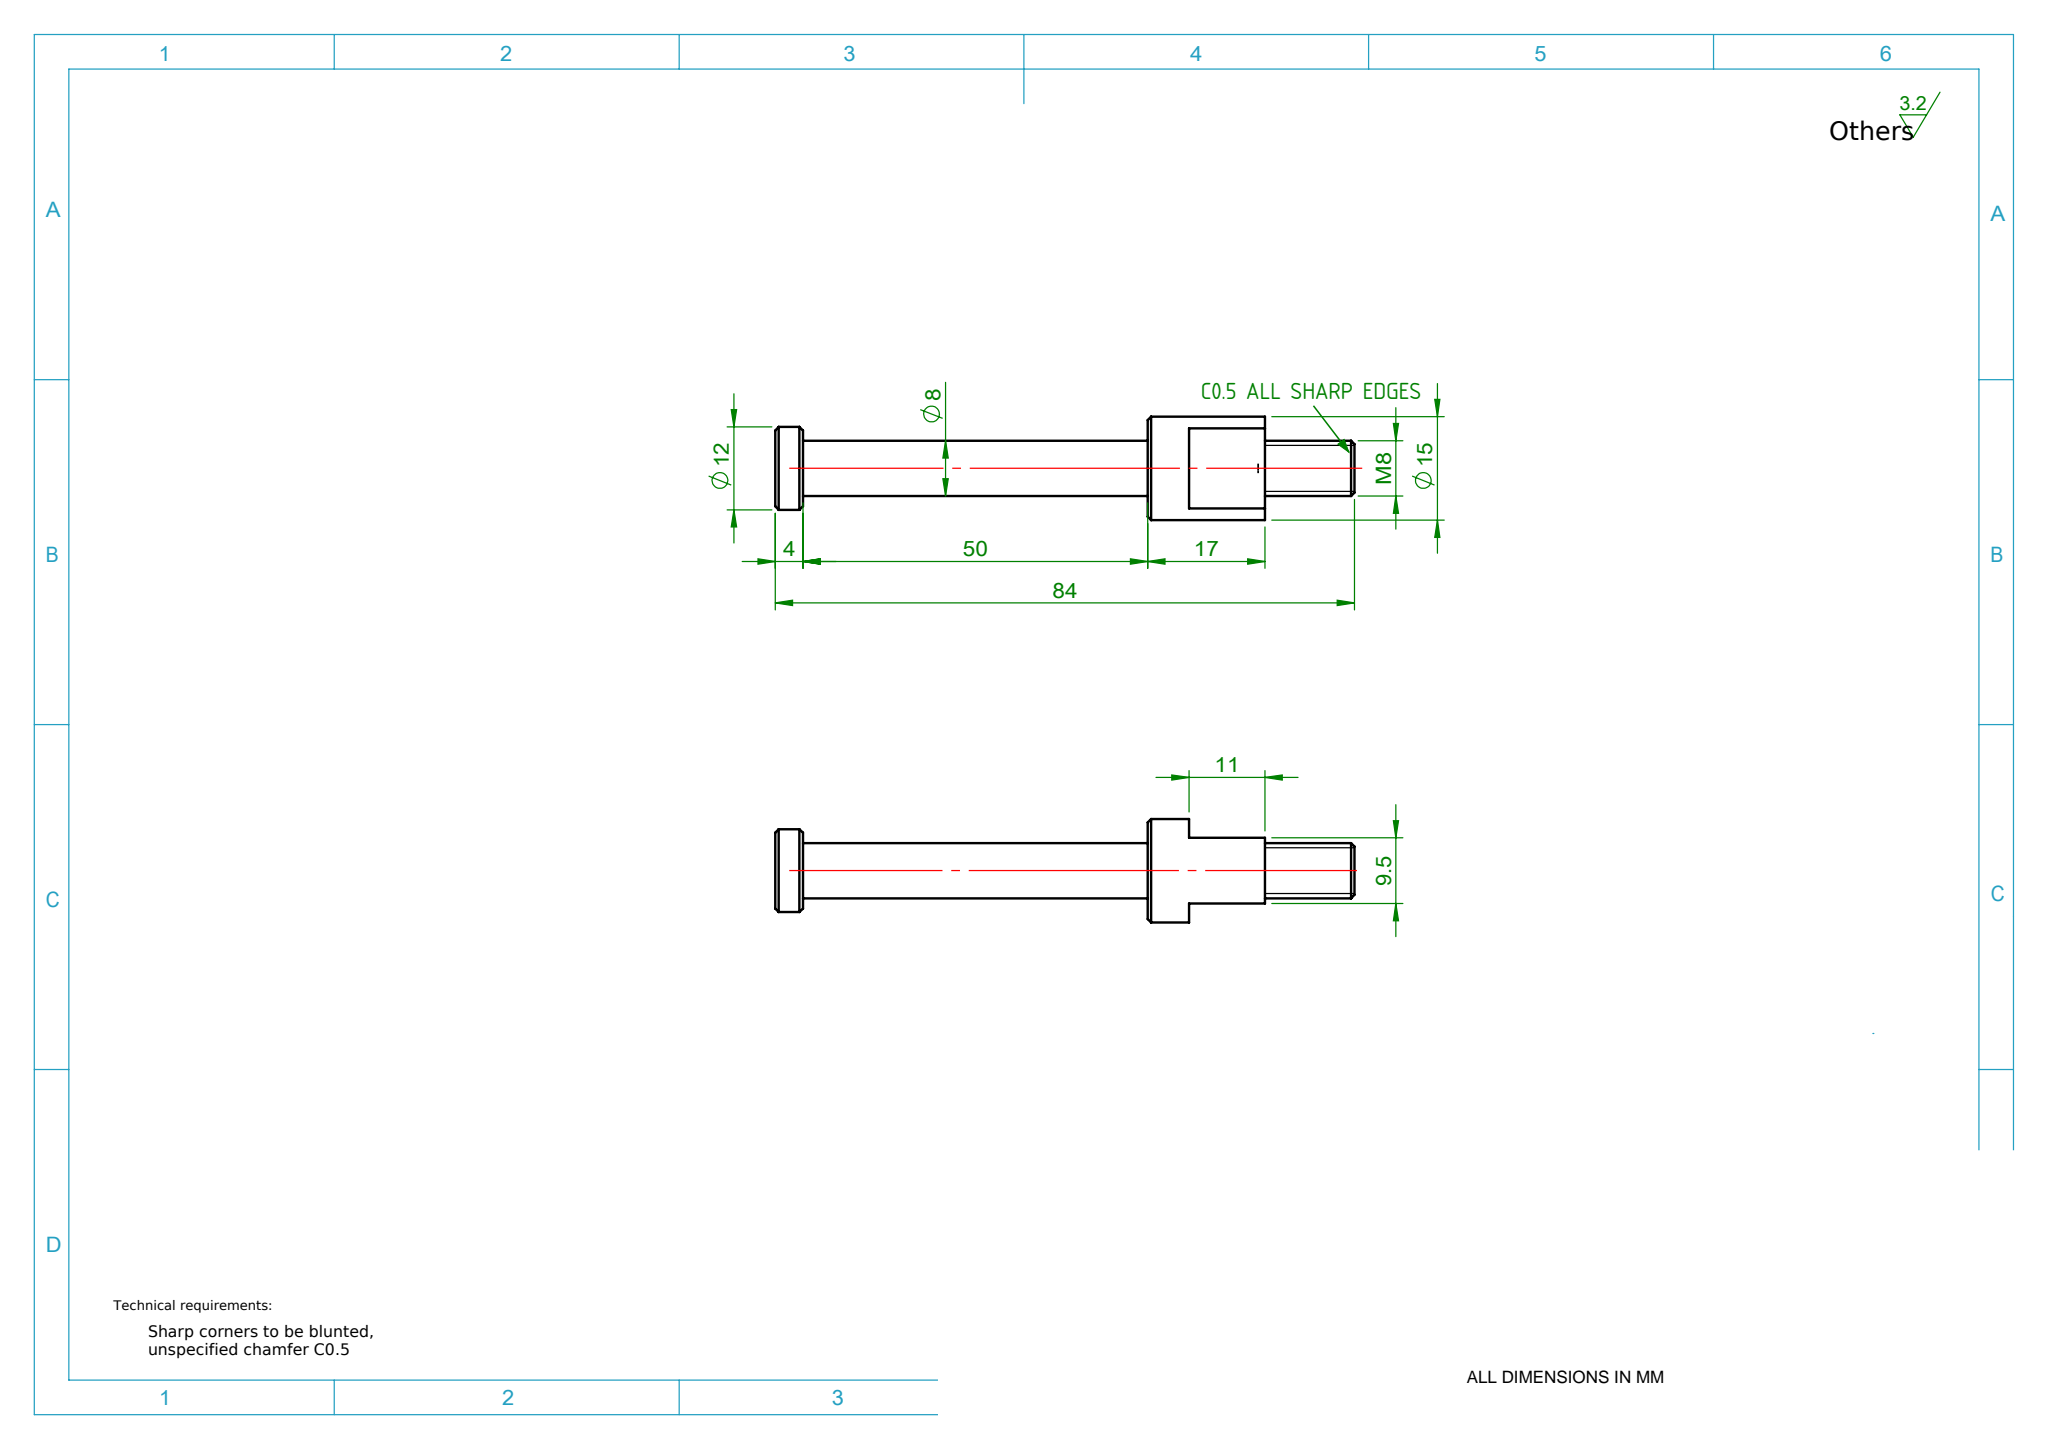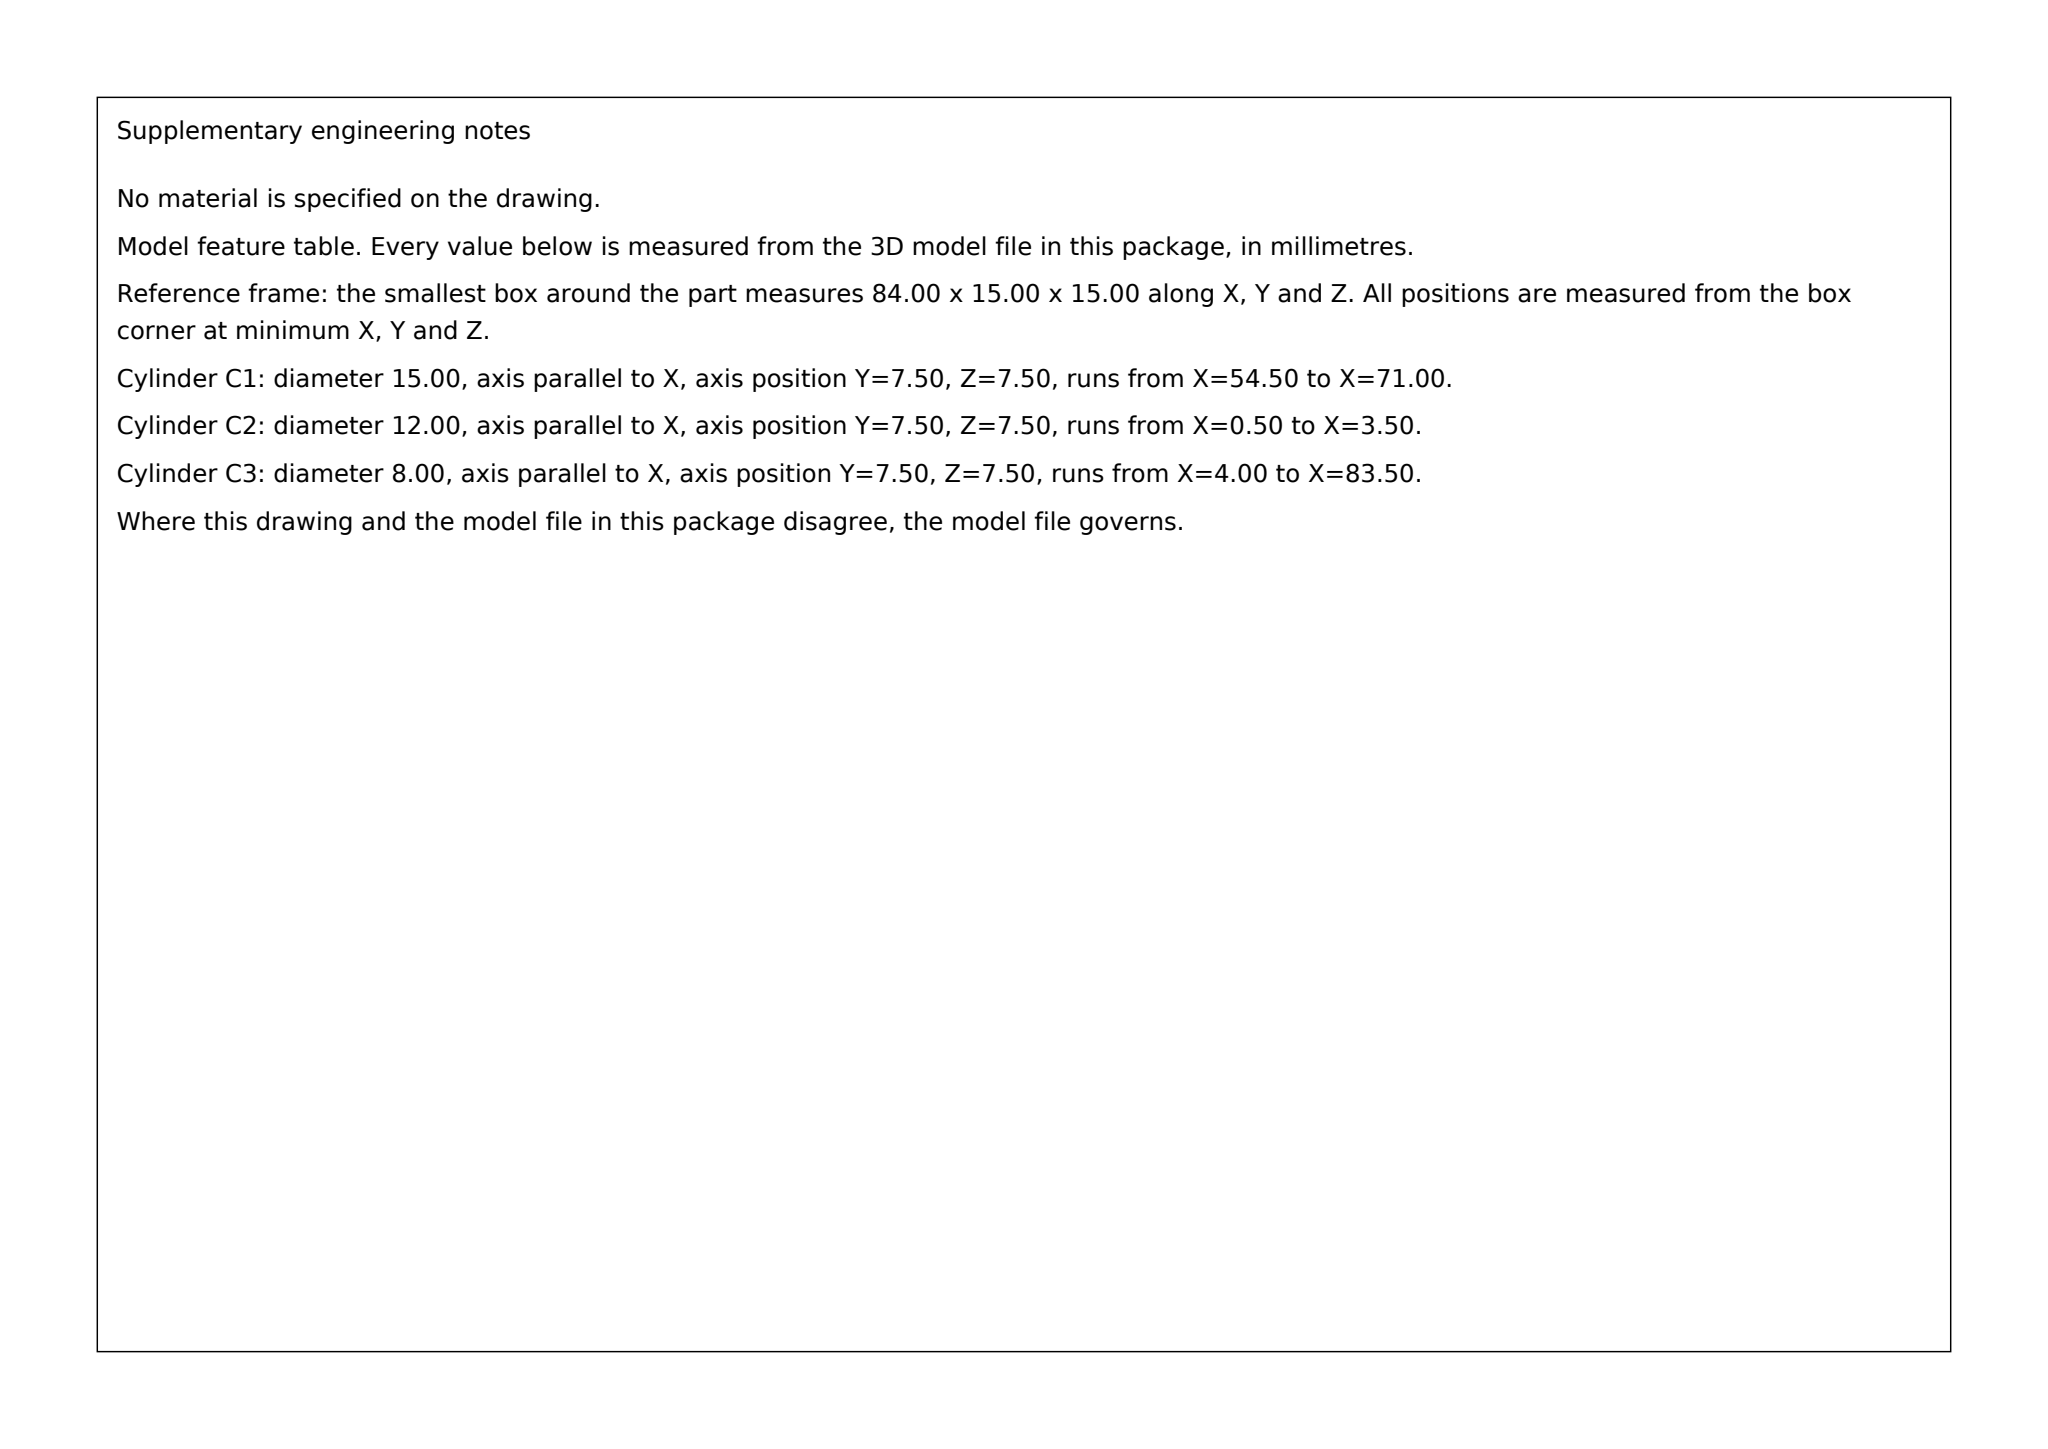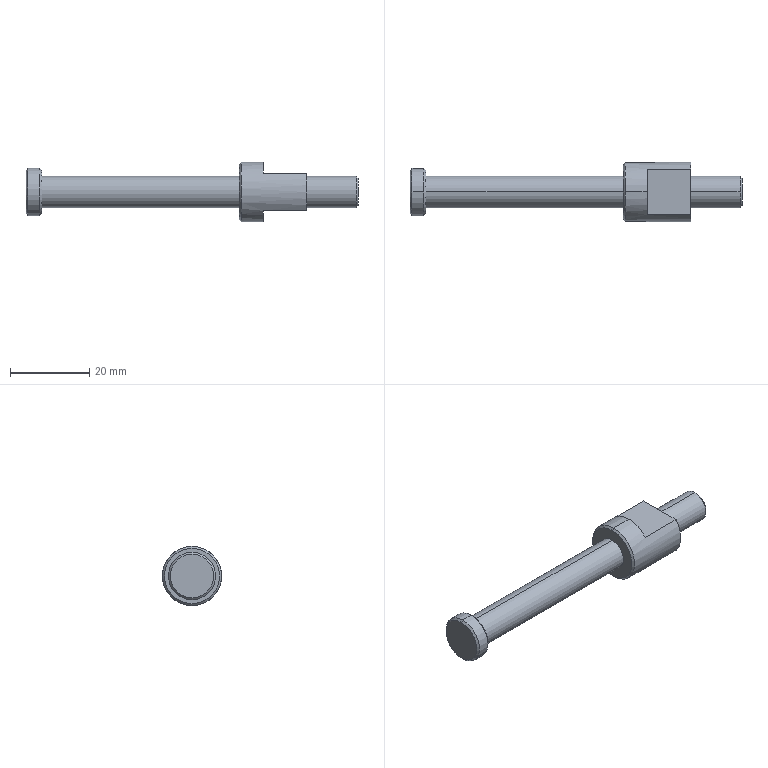Part | SolidWorks | mm | 1 solid | 25 faces | box 84 x 15 x 15 mm | volume 6117 mm3 | plane 9 | cone 8 | cylinder 8 | commonest cylinder face diameters 8 x4 12 x2 15 x2
Drawing notes:
ALL SHARP EDGES C0.5: Ø8, Ø12 & Ø15 ENDS, M8 THREAD END | from the solid: cones[included_angle,ref_dia]: 90°/7 (Ø8), 90°/11 & 12 (Ø12), 90°/14 (Ø15) = 0.5 leg chamfers
build123d program:
from build123d import *

# Parameters (mm, degrees)
SKETCH1_R           = 7.5
BOSS_EXTRUDE1_DEPTH = 84
SKETCH2_R           = 7.5
SKETCH2_R_2         = 6
CUT_EXTRUDE1_DEPTH  = 54
SKETCH3_R           = 6
SKETCH3_R_2         = 4
CUT_EXTRUDE2_DEPTH  = 50
CUT_EXTRUDE3_DEPTH  = 50
CUT_EXTRUDE4_START  = -13
SKETCH5_R           = 10
SKETCH5_R_2         = 4
CUT_EXTRUDE4_DEPTH  = 13
CHAMFER1_SIZE       = 0.5


with BuildPart() as part:
    # Sketch1 → Boss-Extrude1 (new body)
    with BuildSketch(Plane(origin=(0, 0, 0), x_dir=(0, 0, -1), z_dir=(1, 0, 0))):
        with Locations(Location((0, 0, 0), (0, 0, 180))):
            Circle(SKETCH1_R)
    extrude(amount=BOSS_EXTRUDE1_DEPTH)

    # Sketch2 → Cut-Extrude1 (cut)
    with BuildSketch(Plane.ZY):
        Circle(SKETCH2_R)
        Circle(SKETCH2_R_2, mode=Mode.SUBTRACT)
    extrude(amount=-CUT_EXTRUDE1_DEPTH, mode=Mode.SUBTRACT)

    # Sketch3 → Cut-Extrude2 (cut)
    with BuildSketch(Plane.ZY.offset(-4)):
        Circle(SKETCH3_R)
        Circle(SKETCH3_R_2, mode=Mode.SUBTRACT)
    extrude(amount=-CUT_EXTRUDE2_DEPTH, mode=Mode.SUBTRACT)

    # Sketch4 → Cut-Extrude3 (cut)
    with BuildSketch(Plane.ZY.offset(-60)):
        with BuildLine():
            Line((-4.75, 19.428), (-4.75, -19.428))
            ThreePointArc((-4.75, -19.428), (-20, 0), (-4.75, 19.428))
        make_face()
        with BuildLine():
            Line((4.75, 19.428), (4.75, -19.428))
            ThreePointArc((4.75, -19.428), (20, 0), (4.75, 19.428))
        make_face()
    extrude(amount=-CUT_EXTRUDE3_DEPTH, mode=Mode.SUBTRACT)

    # Sketch5 → Cut-Extrude4 (cut)
    with BuildSketch(Plane(origin=(84, 0, 0), x_dir=(0, 0, -1), z_dir=(1, 0, 0)).offset(CUT_EXTRUDE4_START)):
        Circle(SKETCH5_R)
        with Locations(Location((0, 0, 0), (0, 0, 180))):
            Circle(SKETCH5_R_2, mode=Mode.SUBTRACT)
    extrude(amount=CUT_EXTRUDE4_DEPTH, mode=Mode.SUBTRACT)

    # Chamfer1
    chamfer1_edges = [part.edges().sort_by_distance(p)[0] for p in [
        (4, 0, -6),
        (84, 0, -4),
        (54, 0, -7.5),
        (0, 0, -6),
    ]]
    chamfer(chamfer1_edges, length=CHAMFER1_SIZE)


solid = part.part
STEP:
#1=CARTESIAN_POINT('',(0.,0.,5.5));
#2=VERTEX_POINT('',#1);
#3=CARTESIAN_POINT('',(0.,0.,-5.5));
#4=VERTEX_POINT('',#3);
#5=CARTESIAN_POINT('',(0.,0.,0.));
#6=DIRECTION('',(-1.,0.,0.));
#7=DIRECTION('',(0.,0.,-1.));
#8=AXIS2_PLACEMENT_3D('',#5,#6,#7);
#9=CIRCLE('',#8,5.5);
#10=EDGE_CURVE('',#2,#4,#9,.T.);
#11=ORIENTED_EDGE('',*,*,#10,.F.);
#12=CARTESIAN_POINT('',(0.5,0.,6.));
#13=VERTEX_POINT('',#12);
#14=CARTESIAN_POINT('',(0.,0.,5.5));
#15=DIRECTION('',(0.7071,0.,0.7071));
#16=VECTOR('',#15,1000.);
#17=LINE('',#14,#16);
#18=EDGE_CURVE('',#2,#13,#17,.T.);
#19=ORIENTED_EDGE('',*,*,#18,.T.);
#20=CARTESIAN_POINT('',(0.5,0.,-6.));
#21=VERTEX_POINT('',#20);
#22=CARTESIAN_POINT('',(0.5,0.,0.));
#23=DIRECTION('',(1.,0.,0.));
#24=DIRECTION('',(0.,0.,-1.));
#25=AXIS2_PLACEMENT_3D('',#22,#23,#24);
#26=CIRCLE('',#25,6.);
#27=EDGE_CURVE('',#21,#13,#26,.T.);
#28=ORIENTED_EDGE('',*,*,#27,.F.);
#29=CARTESIAN_POINT('',(0.,0.,-5.5));
#30=DIRECTION('',(0.7071,0.,-0.7071));
#31=VECTOR('',#30,1000.);
#32=LINE('',#29,#31);
#33=EDGE_CURVE('',#4,#21,#32,.T.);
#34=ORIENTED_EDGE('',*,*,#33,.F.);
#35=EDGE_LOOP('',(#11,#19,#28,#34));
#36=FACE_OUTER_BOUND('',#35,.T.);
#37=CARTESIAN_POINT('',(0.,0.,0.));
#38=DIRECTION('',(1.,0.,0.));
#39=DIRECTION('',(0.,0.,-1.));
#40=AXIS2_PLACEMENT_3D('',#37,#38,#39);
#41=CONICAL_SURFACE('',#40,5.5,0.7854);
#42=ADVANCED_FACE('',(#36),#41,.T.);
#43=CARTESIAN_POINT('',(4.,0.,-5.5));
#44=VERTEX_POINT('',#43);
#45=CARTESIAN_POINT('',(4.,0.,5.5));
#46=VERTEX_POINT('',#45);
#47=CARTESIAN_POINT('',(4.,0.,0.));
#48=DIRECTION('',(1.,0.,0.));
#49=DIRECTION('',(0.,0.,1.));
#50=AXIS2_PLACEMENT_3D('',#47,#48,#49);
#51=CIRCLE('',#50,5.5);
#52=EDGE_CURVE('',#44,#46,#51,.T.);
#53=ORIENTED_EDGE('',*,*,#52,.F.);
#54=CARTESIAN_POINT('',(3.5,0.,-6.));
#55=VERTEX_POINT('',#54);
#56=CARTESIAN_POINT('',(3.5,0.,-6.));
#57=DIRECTION('',(-0.7071,0.,-0.7071));
#58=VECTOR('',#57,1000.);
#59=LINE('',#56,#58);
#60=EDGE_CURVE('',#44,#55,#59,.T.);
#61=ORIENTED_EDGE('',*,*,#60,.T.);
#62=CARTESIAN_POINT('',(3.5,0.,6.));
#63=VERTEX_POINT('',#62);
#64=CARTESIAN_POINT('',(3.5,0.,0.));
#65=DIRECTION('',(-1.,0.,0.));
#66=DIRECTION('',(0.,0.,1.));
#67=AXIS2_PLACEMENT_3D('',#64,#65,#66);
#68=CIRCLE('',#67,6.);
#69=EDGE_CURVE('',#63,#55,#68,.T.);
#70=ORIENTED_EDGE('',*,*,#69,.F.);
#71=CARTESIAN_POINT('',(3.5,0.,6.));
#72=DIRECTION('',(-0.7071,0.,0.7071));
#73=VECTOR('',#72,1000.);
#74=LINE('',#71,#73);
#75=EDGE_CURVE('',#46,#63,#74,.T.);
#76=ORIENTED_EDGE('',*,*,#75,.F.);
#77=EDGE_LOOP('',(#53,#61,#70,#76));
#78=FACE_OUTER_BOUND('',#77,.T.);
#79=CARTESIAN_POINT('',(3.5,0.,0.));
#80=DIRECTION('',(-1.,0.,0.));
#81=DIRECTION('',(0.,0.,1.));
#82=AXIS2_PLACEMENT_3D('',#79,#80,#81);
#83=CONICAL_SURFACE('',#82,6.,0.7854);
#84=ADVANCED_FACE('',(#78),#83,.T.);
#85=CARTESIAN_POINT('',(54.,0.,7.));
#86=VERTEX_POINT('',#85);
#87=CARTESIAN_POINT('',(54.,0.,-7.));
#88=VERTEX_POINT('',#87);
#89=CARTESIAN_POINT('',(54.,0.,0.));
#90=DIRECTION('',(-1.,0.,0.));
#91=DIRECTION('',(0.,0.,1.));
#92=AXIS2_PLACEMENT_3D('',#89,#90,#91);
#93=CIRCLE('',#92,7.);
#94=EDGE_CURVE('',#86,#88,#93,.T.);
#95=ORIENTED_EDGE('',*,*,#94,.F.);
#96=CARTESIAN_POINT('',(54.5,0.,7.5));
#97=VERTEX_POINT('',#96);
#98=CARTESIAN_POINT('',(54.,0.,7.));
#99=DIRECTION('',(0.7071,0.,0.7071));
#100=VECTOR('',#99,1000.);
#101=LINE('',#98,#100);
#102=EDGE_CURVE('',#86,#97,#101,.T.);
#103=ORIENTED_EDGE('',*,*,#102,.T.);
#104=CARTESIAN_POINT('',(54.5,0.,-7.5));
#105=VERTEX_POINT('',#104);
#106=CARTESIAN_POINT('',(54.5,0.,0.));
#107=DIRECTION('',(1.,0.,0.));
#108=DIRECTION('',(0.,0.,1.));
#109=AXIS2_PLACEMENT_3D('',#106,#107,#108);
#110=CIRCLE('',#109,7.5);
#111=EDGE_CURVE('',#105,#97,#110,.T.);
#112=ORIENTED_EDGE('',*,*,#111,.F.);
#113=CARTESIAN_POINT('',(54.,0.,-7.));
#114=DIRECTION('',(0.7071,0.,-0.7071));
#115=VECTOR('',#114,1000.);
#116=LINE('',#113,#115);
#117=EDGE_CURVE('',#88,#105,#116,.T.);
#118=ORIENTED_EDGE('',*,*,#117,.F.);
#119=EDGE_LOOP('',(#95,#103,#112,#118));
#120=FACE_OUTER_BOUND('',#119,.T.);
#121=CARTESIAN_POINT('',(54.,0.,0.));
#122=DIRECTION('',(1.,0.,0.));
#123=DIRECTION('',(0.,0.,-1.));
#124=AXIS2_PLACEMENT_3D('',#121,#122,#123);
#125=CONICAL_SURFACE('',#124,7.,0.7854);
#126=ADVANCED_FACE('',(#120),#125,.T.);
#127=CARTESIAN_POINT('',(84.,0.,-3.5));
#128=VERTEX_POINT('',#127);
#129=CARTESIAN_POINT('',(84.,0.,3.5));
#130=VERTEX_POINT('',#129);
#131=CARTESIAN_POINT('',(84.,0.,0.));
#132=DIRECTION('',(1.,0.,0.));
#133=DIRECTION('',(0.,0.,-1.));
#134=AXIS2_PLACEMENT_3D('',#131,#132,#133);
#135=CIRCLE('',#134,3.5);
#136=EDGE_CURVE('',#128,#130,#135,.T.);
#137=ORIENTED_EDGE('',*,*,#136,.F.);
#138=CARTESIAN_POINT('',(83.5,0.,-4.));
#139=VERTEX_POINT('',#138);
#140=CARTESIAN_POINT('',(84.,0.,-3.5));
#141=DIRECTION('',(-0.7071,0.,-0.7071));
#142=VECTOR('',#141,1000.);
#143=LINE('',#140,#142);
#144=EDGE_CURVE('',#128,#139,#143,.T.);
#145=ORIENTED_EDGE('',*,*,#144,.T.);
#146=CARTESIAN_POINT('',(83.5,0.,4.));
#147=VERTEX_POINT('',#146);
#148=CARTESIAN_POINT('',(83.5,0.,0.));
#149=DIRECTION('',(-1.,0.,0.));
#150=DIRECTION('',(0.,0.,-1.));
#151=AXIS2_PLACEMENT_3D('',#148,#149,#150);
#152=CIRCLE('',#151,4.);
#153=EDGE_CURVE('',#147,#139,#152,.T.);
#154=ORIENTED_EDGE('',*,*,#153,.F.);
#155=CARTESIAN_POINT('',(84.,0.,3.5));
#156=DIRECTION('',(-0.7071,0.,0.7071));
#157=VECTOR('',#156,1000.);
#158=LINE('',#155,#157);
#159=EDGE_CURVE('',#130,#147,#158,.T.);
#160=ORIENTED_EDGE('',*,*,#159,.F.);
#161=EDGE_LOOP('',(#137,#145,#154,#160));
#162=FACE_OUTER_BOUND('',#161,.T.);
#163=CARTESIAN_POINT('',(84.,0.,0.));
#164=DIRECTION('',(-1.,0.,0.));
#165=DIRECTION('',(0.,0.,1.));
#166=AXIS2_PLACEMENT_3D('',#163,#164,#165);
#167=CONICAL_SURFACE('',#166,3.5,0.7854);
#168=ADVANCED_FACE('',(#162),#167,.T.);
#169=CARTESIAN_POINT('',(71.,0.,-4.));
#170=VERTEX_POINT('',#169);
#171=CARTESIAN_POINT('',(71.,0.,4.));
#172=VERTEX_POINT('',#171);
#173=CARTESIAN_POINT('',(71.,0.,0.));
#174=DIRECTION('',(1.,0.,0.));
#175=DIRECTION('',(0.,0.,-1.));
#176=AXIS2_PLACEMENT_3D('',#173,#174,#175);
#177=CIRCLE('',#176,4.);
#178=EDGE_CURVE('',#170,#172,#177,.T.);
#179=ORIENTED_EDGE('',*,*,#178,.T.);
#180=CARTESIAN_POINT('',(71.,0.,4.));
#181=DIRECTION('',(1.,0.,0.));
#182=VECTOR('',#181,1000.);
#183=LINE('',#180,#182);
#184=EDGE_CURVE('',#172,#147,#183,.T.);
#185=ORIENTED_EDGE('',*,*,#184,.T.);
#186=ORIENTED_EDGE('',*,*,#153,.T.);
#187=CARTESIAN_POINT('',(71.,0.,-4.));
#188=DIRECTION('',(1.,0.,0.));
#189=VECTOR('',#188,1000.);
#190=LINE('',#187,#189);
#191=EDGE_CURVE('',#170,#139,#190,.T.);
#192=ORIENTED_EDGE('',*,*,#191,.F.);
#193=EDGE_LOOP('',(#179,#185,#186,#192));
#194=FACE_OUTER_BOUND('',#193,.T.);
#195=CARTESIAN_POINT('',(71.,0.,0.));
#196=DIRECTION('',(1.,0.,0.));
#197=DIRECTION('',(0.,0.,-1.));
#198=AXIS2_PLACEMENT_3D('',#195,#196,#197);
#199=CYLINDRICAL_SURFACE('',#198,4.);
#200=ADVANCED_FACE('',(#194),#199,.T.);
#201=ORIENTED_EDGE('',*,*,#69,.T.);
#202=CARTESIAN_POINT('',(54.,0.,-6.));
#203=DIRECTION('',(-1.,0.,0.));
#204=VECTOR('',#203,1000.);
#205=LINE('',#202,#204);
#206=EDGE_CURVE('',#55,#21,#205,.T.);
#207=ORIENTED_EDGE('',*,*,#206,.T.);
#208=ORIENTED_EDGE('',*,*,#27,.T.);
#209=CARTESIAN_POINT('',(54.,0.,6.));
#210=DIRECTION('',(-1.,0.,0.));
#211=VECTOR('',#210,1000.);
#212=LINE('',#209,#211);
#213=EDGE_CURVE('',#63,#13,#212,.T.);
#214=ORIENTED_EDGE('',*,*,#213,.F.);
#215=EDGE_LOOP('',(#201,#207,#208,#214));
#216=FACE_OUTER_BOUND('',#215,.T.);
#217=CARTESIAN_POINT('',(54.,0.,0.));
#218=DIRECTION('',(-1.,0.,0.));
#219=DIRECTION('',(0.,0.,1.));
#220=AXIS2_PLACEMENT_3D('',#217,#218,#219);
#221=CYLINDRICAL_SURFACE('',#220,6.);
#222=ADVANCED_FACE('',(#216),#221,.T.);
#223=CARTESIAN_POINT('',(54.,0.,4.));
#224=VERTEX_POINT('',#223);
#225=CARTESIAN_POINT('',(54.,0.,-4.));
#226=VERTEX_POINT('',#225);
#227=CARTESIAN_POINT('',(54.,0.,0.));
#228=DIRECTION('',(-1.,0.,0.));
#229=DIRECTION('',(0.,0.,1.));
#230=AXIS2_PLACEMENT_3D('',#227,#228,#229);
#231=CIRCLE('',#230,4.);
#232=EDGE_CURVE('',#224,#226,#231,.T.);
#233=ORIENTED_EDGE('',*,*,#232,.T.);
#234=CARTESIAN_POINT('',(4.,0.,-4.));
#235=VERTEX_POINT('',#234);
#236=CARTESIAN_POINT('',(54.,0.,-4.));
#237=DIRECTION('',(-1.,0.,0.));
#238=VECTOR('',#237,1000.);
#239=LINE('',#236,#238);
#240=EDGE_CURVE('',#226,#235,#239,.T.);
#241=ORIENTED_EDGE('',*,*,#240,.T.);
#242=CARTESIAN_POINT('',(4.,0.,4.));
#243=VERTEX_POINT('',#242);
#244=CARTESIAN_POINT('',(4.,0.,0.));
#245=DIRECTION('',(-1.,0.,0.));
#246=DIRECTION('',(0.,0.,1.));
#247=AXIS2_PLACEMENT_3D('',#244,#245,#246);
#248=CIRCLE('',#247,4.);
#249=EDGE_CURVE('',#243,#235,#248,.T.);
#250=ORIENTED_EDGE('',*,*,#249,.F.);
#251=CARTESIAN_POINT('',(54.,0.,4.));
#252=DIRECTION('',(-1.,0.,0.));
#253=VECTOR('',#252,1000.);
#254=LINE('',#251,#253);
#255=EDGE_CURVE('',#224,#243,#254,.T.);
#256=ORIENTED_EDGE('',*,*,#255,.F.);
#257=EDGE_LOOP('',(#233,#241,#250,#256));
#258=FACE_OUTER_BOUND('',#257,.T.);
#259=CARTESIAN_POINT('',(54.,0.,0.));
#260=DIRECTION('',(-1.,0.,0.));
#261=DIRECTION('',(0.,0.,1.));
#262=AXIS2_PLACEMENT_3D('',#259,#260,#261);
#263=CYLINDRICAL_SURFACE('',#262,4.);
#264=ADVANCED_FACE('',(#258),#263,.T.);
#265=CARTESIAN_POINT('',(60.,5.804,-4.75));
#266=VERTEX_POINT('',#265);
#267=CARTESIAN_POINT('',(60.,0.,-7.5));
#268=VERTEX_POINT('',#267);
#269=CARTESIAN_POINT('',(60.,0.,0.));
#270=DIRECTION('',(-1.,0.,0.));
#271=DIRECTION('',(0.,0.,1.));
#272=AXIS2_PLACEMENT_3D('',#269,#270,#271);
#273=CIRCLE('',#272,7.5);
#274=EDGE_CURVE('',#266,#268,#273,.T.);
#275=ORIENTED_EDGE('',*,*,#274,.T.);
#276=CARTESIAN_POINT('',(84.,0.,-7.5));
#277=DIRECTION('',(-1.,0.,0.));
#278=VECTOR('',#277,1000.);
#279=LINE('',#276,#278);
#280=EDGE_CURVE('',#268,#105,#279,.T.);
#281=ORIENTED_EDGE('',*,*,#280,.T.);
#282=ORIENTED_EDGE('',*,*,#111,.T.);
#283=CARTESIAN_POINT('',(60.,0.,7.5));
#284=VERTEX_POINT('',#283);
#285=CARTESIAN_POINT('',(84.,0.,7.5));
#286=DIRECTION('',(-1.,0.,0.));
#287=VECTOR('',#286,1000.);
#288=LINE('',#285,#287);
#289=EDGE_CURVE('',#284,#97,#288,.T.);
#290=ORIENTED_EDGE('',*,*,#289,.F.);
#291=CARTESIAN_POINT('',(60.,5.804,4.75));
#292=VERTEX_POINT('',#291);
#293=CARTESIAN_POINT('',(60.,0.,0.));
#294=DIRECTION('',(-1.,0.,0.));
#295=DIRECTION('',(0.,0.,1.));
#296=AXIS2_PLACEMENT_3D('',#293,#294,#295);
#297=CIRCLE('',#296,7.5);
#298=EDGE_CURVE('',#284,#292,#297,.T.);
#299=ORIENTED_EDGE('',*,*,#298,.T.);
#300=CARTESIAN_POINT('',(71.,5.804,4.75));
#301=VERTEX_POINT('',#300);
#302=CARTESIAN_POINT('',(84.,5.804,4.75));
#303=DIRECTION('',(1.,0.,0.));
#304=VECTOR('',#303,1000.);
#305=LINE('',#302,#304);
#306=EDGE_CURVE('',#292,#301,#305,.T.);
#307=ORIENTED_EDGE('',*,*,#306,.T.);
#308=CARTESIAN_POINT('',(71.,5.804,-4.75));
#309=VERTEX_POINT('',#308);
#310=CARTESIAN_POINT('',(71.,0.,0.));
#311=DIRECTION('',(1.,0.,0.));
#312=DIRECTION('',(0.,0.,-1.));
#313=AXIS2_PLACEMENT_3D('',#310,#311,#312);
#314=CIRCLE('',#313,7.5);
#315=EDGE_CURVE('',#309,#301,#314,.T.);
#316=ORIENTED_EDGE('',*,*,#315,.F.);
#317=CARTESIAN_POINT('',(84.,5.804,-4.75));
#318=DIRECTION('',(-1.,0.,0.));
#319=VECTOR('',#318,1000.);
#320=LINE('',#317,#319);
#321=EDGE_CURVE('',#309,#266,#320,.T.);
#322=ORIENTED_EDGE('',*,*,#321,.T.);
#323=EDGE_LOOP('',(#275,#281,#282,#290,#299,#307,#316,#322));
#324=FACE_OUTER_BOUND('',#323,.T.);
#325=CARTESIAN_POINT('',(84.,0.,0.));
#326=DIRECTION('',(-1.,0.,0.));
#327=DIRECTION('',(0.,0.,1.));
#328=AXIS2_PLACEMENT_3D('',#325,#326,#327);
#329=CYLINDRICAL_SURFACE('',#328,7.5);
#330=ADVANCED_FACE('',(#324),#329,.T.);
#331=ORIENTED_EDGE('',*,*,#280,.F.);
#332=CARTESIAN_POINT('',(60.,-5.804,-4.75));
#333=VERTEX_POINT('',#332);
#334=CARTESIAN_POINT('',(60.,0.,0.));
#335=DIRECTION('',(-1.,0.,0.));
#336=DIRECTION('',(0.,0.,1.));
#337=AXIS2_PLACEMENT_3D('',#334,#335,#336);
#338=CIRCLE('',#337,7.5);
#339=EDGE_CURVE('',#268,#333,#338,.T.);
#340=ORIENTED_EDGE('',*,*,#339,.T.);
#341=CARTESIAN_POINT('',(71.,-5.804,-4.75));
#342=VERTEX_POINT('',#341);
#343=CARTESIAN_POINT('',(84.,-5.804,-4.75));
#344=DIRECTION('',(1.,0.,0.));
#345=VECTOR('',#344,1000.);
#346=LINE('',#343,#345);
#347=EDGE_CURVE('',#333,#342,#346,.T.);
#348=ORIENTED_EDGE('',*,*,#347,.T.);
#349=CARTESIAN_POINT('',(71.,-5.804,4.75));
#350=VERTEX_POINT('',#349);
#351=CARTESIAN_POINT('',(71.,0.,0.));
#352=DIRECTION('',(1.,0.,0.));
#353=DIRECTION('',(0.,0.,-1.));
#354=AXIS2_PLACEMENT_3D('',#351,#352,#353);
#355=CIRCLE('',#354,7.5);
#356=EDGE_CURVE('',#350,#342,#355,.T.);
#357=ORIENTED_EDGE('',*,*,#356,.F.);
#358=CARTESIAN_POINT('',(60.,-5.804,4.75));
#359=VERTEX_POINT('',#358);
#360=CARTESIAN_POINT('',(84.,-5.804,4.75));
#361=DIRECTION('',(-1.,0.,0.));
#362=VECTOR('',#361,1000.);
#363=LINE('',#360,#362);
#364=EDGE_CURVE('',#350,#359,#363,.T.);
#365=ORIENTED_EDGE('',*,*,#364,.T.);
#366=CARTESIAN_POINT('',(60.,0.,0.));
#367=DIRECTION('',(-1.,0.,0.));
#368=DIRECTION('',(0.,0.,1.));
#369=AXIS2_PLACEMENT_3D('',#366,#367,#368);
#370=CIRCLE('',#369,7.5);
#371=EDGE_CURVE('',#359,#284,#370,.T.);
#372=ORIENTED_EDGE('',*,*,#371,.T.);
#373=ORIENTED_EDGE('',*,*,#289,.T.);
#374=CARTESIAN_POINT('',(54.5,0.,0.));
#375=DIRECTION('',(1.,0.,0.));
#376=DIRECTION('',(0.,0.,1.));
#377=AXIS2_PLACEMENT_3D('',#374,#375,#376);
#378=CIRCLE('',#377,7.5);
#379=EDGE_CURVE('',#97,#105,#378,.T.);
#380=ORIENTED_EDGE('',*,*,#379,.T.);
#381=EDGE_LOOP('',(#331,#340,#348,#357,#365,#372,#373,#380));
#382=FACE_OUTER_BOUND('',#381,.T.);
#383=CARTESIAN_POINT('',(84.,0.,0.));
#384=DIRECTION('',(-1.,0.,0.));
#385=DIRECTION('',(0.,0.,1.));
#386=AXIS2_PLACEMENT_3D('',#383,#384,#385);
#387=CYLINDRICAL_SURFACE('',#386,7.5);
#388=ADVANCED_FACE('',(#382),#387,.T.);
#389=CARTESIAN_POINT('',(71.,19.428,4.75));
#390=DIRECTION('',(0.,-1.,0.));
#391=VECTOR('',#390,1000.);
#392=LINE('',#389,#391);
#393=EDGE_CURVE('',#301,#350,#392,.T.);
#394=ORIENTED_EDGE('',*,*,#393,.F.);
#395=ORIENTED_EDGE('',*,*,#306,.F.);
#396=CARTESIAN_POINT('',(60.,19.428,4.75));
#397=DIRECTION('',(0.,-1.,0.));
#398=VECTOR('',#397,1000.);
#399=LINE('',#396,#398);
#400=EDGE_CURVE('',#292,#359,#399,.T.);
#401=ORIENTED_EDGE('',*,*,#400,.T.);
#402=ORIENTED_EDGE('',*,*,#364,.F.);
#403=EDGE_LOOP('',(#394,#395,#401,#402));
#404=FACE_OUTER_BOUND('',#403,.T.);
#405=CARTESIAN_POINT('',(110.,19.428,4.75));
#406=DIRECTION('',(0.,0.,-1.));
#407=DIRECTION('',(-1.,0.,0.));
#408=AXIS2_PLACEMENT_3D('',#405,#406,#407);
#409=PLANE('',#408);
#410=ADVANCED_FACE('',(#404),#409,.F.);
#411=CARTESIAN_POINT('',(71.,19.428,-4.75));
#412=DIRECTION('',(0.,1.,0.));
#413=VECTOR('',#412,1000.);
#414=LINE('',#411,#413);
#415=EDGE_CURVE('',#342,#309,#414,.T.);
#416=ORIENTED_EDGE('',*,*,#415,.F.);
#417=ORIENTED_EDGE('',*,*,#347,.F.);
#418=CARTESIAN_POINT('',(60.,19.428,-4.75));
#419=DIRECTION('',(0.,1.,0.));
#420=VECTOR('',#419,1000.);
#421=LINE('',#418,#420);
#422=EDGE_CURVE('',#333,#266,#421,.T.);
#423=ORIENTED_EDGE('',*,*,#422,.T.);
#424=ORIENTED_EDGE('',*,*,#321,.F.);
#425=EDGE_LOOP('',(#416,#417,#423,#424));
#426=FACE_OUTER_BOUND('',#425,.T.);
#427=CARTESIAN_POINT('',(110.,19.428,-4.75));
#428=DIRECTION('',(0.,0.,1.));
#429=DIRECTION('',(1.,0.,0.));
#430=AXIS2_PLACEMENT_3D('',#427,#428,#429);
#431=PLANE('',#430);
#432=ADVANCED_FACE('',(#426),#431,.F.);
#433=CARTESIAN_POINT('',(54.,0.,0.));
#434=DIRECTION('',(-1.,0.,0.));
#435=DIRECTION('',(0.,0.,1.));
#436=AXIS2_PLACEMENT_3D('',#433,#434,#435);
#437=CIRCLE('',#436,7.);
#438=EDGE_CURVE('',#88,#86,#437,.T.);
#439=ORIENTED_EDGE('',*,*,#438,.T.);
#440=ORIENTED_EDGE('',*,*,#94,.T.);
#441=EDGE_LOOP('',(#439,#440));
#442=FACE_OUTER_BOUND('',#441,.T.);
#443=ORIENTED_EDGE('',*,*,#232,.F.);
#444=CARTESIAN_POINT('',(54.,0.,0.));
#445=DIRECTION('',(-1.,0.,0.));
#446=DIRECTION('',(0.,0.,1.));
#447=AXIS2_PLACEMENT_3D('',#444,#445,#446);
#448=CIRCLE('',#447,4.);
#449=EDGE_CURVE('',#226,#224,#448,.T.);
#450=ORIENTED_EDGE('',*,*,#449,.F.);
#451=EDGE_LOOP('',(#443,#450));
#452=FACE_BOUND('',#451,.T.);
#453=CARTESIAN_POINT('',(54.,0.,0.));
#454=DIRECTION('',(-1.,0.,0.));
#455=DIRECTION('',(0.,0.,1.));
#456=AXIS2_PLACEMENT_3D('',#453,#454,#455);
#457=PLANE('',#456);
#458=ADVANCED_FACE('',(#442,#452),#457,.T.);
#459=CARTESIAN_POINT('',(4.,0.,0.));
#460=DIRECTION('',(1.,0.,0.));
#461=DIRECTION('',(0.,0.,1.));
#462=AXIS2_PLACEMENT_3D('',#459,#460,#461);
#463=CIRCLE('',#462,5.5);
#464=EDGE_CURVE('',#46,#44,#463,.T.);
#465=ORIENTED_EDGE('',*,*,#464,.T.);
#466=ORIENTED_EDGE('',*,*,#52,.T.);
#467=EDGE_LOOP('',(#465,#466));
#468=FACE_OUTER_BOUND('',#467,.T.);
#469=ORIENTED_EDGE('',*,*,#249,.T.);
#470=CARTESIAN_POINT('',(4.,0.,0.));
#471=DIRECTION('',(-1.,0.,0.));
#472=DIRECTION('',(0.,0.,1.));
#473=AXIS2_PLACEMENT_3D('',#470,#471,#472);
#474=CIRCLE('',#473,4.);
#475=EDGE_CURVE('',#235,#243,#474,.T.);
#476=ORIENTED_EDGE('',*,*,#475,.T.);
#477=EDGE_LOOP('',(#469,#476));
#478=FACE_BOUND('',#477,.T.);
#479=CARTESIAN_POINT('',(4.,0.,0.));
#480=DIRECTION('',(-1.,0.,0.));
#481=DIRECTION('',(0.,0.,1.));
#482=AXIS2_PLACEMENT_3D('',#479,#480,#481);
#483=PLANE('',#482);
#484=ADVANCED_FACE('',(#468,#478),#483,.F.);
#485=ORIENTED_EDGE('',*,*,#240,.F.);
#486=ORIENTED_EDGE('',*,*,#449,.T.);
#487=ORIENTED_EDGE('',*,*,#255,.T.);
#488=ORIENTED_EDGE('',*,*,#475,.F.);
#489=EDGE_LOOP('',(#485,#486,#487,#488));
#490=FACE_OUTER_BOUND('',#489,.T.);
#491=CARTESIAN_POINT('',(54.,0.,0.));
#492=DIRECTION('',(-1.,0.,0.));
#493=DIRECTION('',(0.,0.,1.));
#494=AXIS2_PLACEMENT_3D('',#491,#492,#493);
#495=CYLINDRICAL_SURFACE('',#494,4.);
#496=ADVANCED_FACE('',(#490),#495,.T.);
#497=CARTESIAN_POINT('',(0.,0.,0.));
#498=DIRECTION('',(-1.,0.,0.));
#499=DIRECTION('',(0.,0.,-1.));
#500=AXIS2_PLACEMENT_3D('',#497,#498,#499);
#501=CIRCLE('',#500,5.5);
#502=EDGE_CURVE('',#4,#2,#501,.T.);
#503=ORIENTED_EDGE('',*,*,#502,.T.);
#504=ORIENTED_EDGE('',*,*,#10,.T.);
#505=EDGE_LOOP('',(#503,#504));
#506=FACE_OUTER_BOUND('',#505,.T.);
#507=CARTESIAN_POINT('',(0.,0.,0.));
#508=DIRECTION('',(1.,0.,0.));
#509=DIRECTION('',(0.,0.,-1.));
#510=AXIS2_PLACEMENT_3D('',#507,#508,#509);
#511=PLANE('',#510);
#512=ADVANCED_FACE('',(#506),#511,.F.);
#513=ORIENTED_EDGE('',*,*,#206,.F.);
#514=CARTESIAN_POINT('',(3.5,0.,0.));
#515=DIRECTION('',(-1.,0.,0.));
#516=DIRECTION('',(0.,0.,1.));
#517=AXIS2_PLACEMENT_3D('',#514,#515,#516);
#518=CIRCLE('',#517,6.);
#519=EDGE_CURVE('',#55,#63,#518,.T.);
#520=ORIENTED_EDGE('',*,*,#519,.T.);
#521=ORIENTED_EDGE('',*,*,#213,.T.);
#522=CARTESIAN_POINT('',(0.5,0.,0.));
#523=DIRECTION('',(1.,0.,0.));
#524=DIRECTION('',(0.,0.,-1.));
#525=AXIS2_PLACEMENT_3D('',#522,#523,#524);
#526=CIRCLE('',#525,6.);
#527=EDGE_CURVE('',#13,#21,#526,.T.);
#528=ORIENTED_EDGE('',*,*,#527,.T.);
#529=EDGE_LOOP('',(#513,#520,#521,#528));
#530=FACE_OUTER_BOUND('',#529,.T.);
#531=CARTESIAN_POINT('',(54.,0.,0.));
#532=DIRECTION('',(-1.,0.,0.));
#533=DIRECTION('',(0.,0.,1.));
#534=AXIS2_PLACEMENT_3D('',#531,#532,#533);
#535=CYLINDRICAL_SURFACE('',#534,6.);
#536=ADVANCED_FACE('',(#530),#535,.T.);
#537=ORIENTED_EDGE('',*,*,#400,.F.);
#538=ORIENTED_EDGE('',*,*,#298,.F.);
#539=ORIENTED_EDGE('',*,*,#371,.F.);
#540=EDGE_LOOP('',(#537,#538,#539));
#541=FACE_OUTER_BOUND('',#540,.T.);
#542=CARTESIAN_POINT('',(60.,0.,0.));
#543=DIRECTION('',(-1.,0.,0.));
#544=DIRECTION('',(0.,0.,1.));
#545=AXIS2_PLACEMENT_3D('',#542,#543,#544);
#546=PLANE('',#545);
#547=ADVANCED_FACE('',(#541),#546,.F.);
#548=ORIENTED_EDGE('',*,*,#422,.F.);
#549=ORIENTED_EDGE('',*,*,#339,.F.);
#550=ORIENTED_EDGE('',*,*,#274,.F.);
#551=EDGE_LOOP('',(#548,#549,#550));
#552=FACE_OUTER_BOUND('',#551,.T.);
#553=CARTESIAN_POINT('',(60.,0.,0.));
#554=DIRECTION('',(-1.,0.,0.));
#555=DIRECTION('',(0.,0.,1.));
#556=AXIS2_PLACEMENT_3D('',#553,#554,#555);
#557=PLANE('',#556);
#558=ADVANCED_FACE('',(#552),#557,.F.);
#559=ORIENTED_EDGE('',*,*,#178,.F.);
#560=CARTESIAN_POINT('',(71.,0.,0.));
#561=DIRECTION('',(1.,0.,0.));
#562=DIRECTION('',(0.,0.,-1.));
#563=AXIS2_PLACEMENT_3D('',#560,#561,#562);
#564=CIRCLE('',#563,4.);
#565=EDGE_CURVE('',#172,#170,#564,.T.);
#566=ORIENTED_EDGE('',*,*,#565,.F.);
#567=EDGE_LOOP('',(#559,#566));
#568=FACE_BOUND('',#567,.T.);
#569=ORIENTED_EDGE('',*,*,#393,.T.);
#570=ORIENTED_EDGE('',*,*,#356,.T.);
#571=ORIENTED_EDGE('',*,*,#415,.T.);
#572=ORIENTED_EDGE('',*,*,#315,.T.);
#573=EDGE_LOOP('',(#569,#570,#571,#572));
#574=FACE_OUTER_BOUND('',#573,.T.);
#575=CARTESIAN_POINT('',(71.,0.,0.));
#576=DIRECTION('',(1.,0.,0.));
#577=DIRECTION('',(0.,0.,-1.));
#578=AXIS2_PLACEMENT_3D('',#575,#576,#577);
#579=PLANE('',#578);
#580=ADVANCED_FACE('',(#568,#574),#579,.T.);
#581=ORIENTED_EDGE('',*,*,#184,.F.);
#582=ORIENTED_EDGE('',*,*,#565,.T.);
#583=ORIENTED_EDGE('',*,*,#191,.T.);
#584=CARTESIAN_POINT('',(83.5,0.,0.));
#585=DIRECTION('',(-1.,0.,0.));
#586=DIRECTION('',(0.,0.,-1.));
#587=AXIS2_PLACEMENT_3D('',#584,#585,#586);
#588=CIRCLE('',#587,4.);
#589=EDGE_CURVE('',#139,#147,#588,.T.);
#590=ORIENTED_EDGE('',*,*,#589,.T.);
#591=EDGE_LOOP('',(#581,#582,#583,#590));
#592=FACE_OUTER_BOUND('',#591,.T.);
#593=CARTESIAN_POINT('',(71.,0.,0.));
#594=DIRECTION('',(1.,0.,0.));
#595=DIRECTION('',(0.,0.,-1.));
#596=AXIS2_PLACEMENT_3D('',#593,#594,#595);
#597=CYLINDRICAL_SURFACE('',#596,4.);
#598=ADVANCED_FACE('',(#592),#597,.T.);
#599=CARTESIAN_POINT('',(84.,0.,0.));
#600=DIRECTION('',(1.,0.,0.));
#601=DIRECTION('',(0.,0.,-1.));
#602=AXIS2_PLACEMENT_3D('',#599,#600,#601);
#603=CIRCLE('',#602,3.5);
#604=EDGE_CURVE('',#130,#128,#603,.T.);
#605=ORIENTED_EDGE('',*,*,#604,.T.);
#606=ORIENTED_EDGE('',*,*,#136,.T.);
#607=EDGE_LOOP('',(#605,#606));
#608=FACE_OUTER_BOUND('',#607,.T.);
#609=CARTESIAN_POINT('',(84.,0.,0.));
#610=DIRECTION('',(1.,0.,0.));
#611=DIRECTION('',(0.,0.,-1.));
#612=AXIS2_PLACEMENT_3D('',#609,#610,#611);
#613=PLANE('',#612);
#614=ADVANCED_FACE('',(#608),#613,.T.);
#615=ORIENTED_EDGE('',*,*,#144,.F.);
#616=ORIENTED_EDGE('',*,*,#604,.F.);
#617=ORIENTED_EDGE('',*,*,#159,.T.);
#618=ORIENTED_EDGE('',*,*,#589,.F.);
#619=EDGE_LOOP('',(#615,#616,#617,#618));
#620=FACE_OUTER_BOUND('',#619,.T.);
#621=CARTESIAN_POINT('',(84.,0.,0.));
#622=DIRECTION('',(-1.,0.,0.));
#623=DIRECTION('',(0.,0.,1.));
#624=AXIS2_PLACEMENT_3D('',#621,#622,#623);
#625=CONICAL_SURFACE('',#624,3.5,0.7854);
#626=ADVANCED_FACE('',(#620),#625,.T.);
#627=ORIENTED_EDGE('',*,*,#102,.F.);
#628=ORIENTED_EDGE('',*,*,#438,.F.);
#629=ORIENTED_EDGE('',*,*,#117,.T.);
#630=ORIENTED_EDGE('',*,*,#379,.F.);
#631=EDGE_LOOP('',(#627,#628,#629,#630));
#632=FACE_OUTER_BOUND('',#631,.T.);
#633=CARTESIAN_POINT('',(54.,0.,0.));
#634=DIRECTION('',(1.,0.,0.));
#635=DIRECTION('',(0.,0.,-1.));
#636=AXIS2_PLACEMENT_3D('',#633,#634,#635);
#637=CONICAL_SURFACE('',#636,7.,0.7854);
#638=ADVANCED_FACE('',(#632),#637,.T.);
#639=ORIENTED_EDGE('',*,*,#60,.F.);
#640=ORIENTED_EDGE('',*,*,#464,.F.);
#641=ORIENTED_EDGE('',*,*,#75,.T.);
#642=ORIENTED_EDGE('',*,*,#519,.F.);
#643=EDGE_LOOP('',(#639,#640,#641,#642));
#644=FACE_OUTER_BOUND('',#643,.T.);
#645=CARTESIAN_POINT('',(3.5,0.,0.));
#646=DIRECTION('',(-1.,0.,0.));
#647=DIRECTION('',(0.,0.,1.));
#648=AXIS2_PLACEMENT_3D('',#645,#646,#647);
#649=CONICAL_SURFACE('',#648,6.,0.7854);
#650=ADVANCED_FACE('',(#644),#649,.T.);
#651=ORIENTED_EDGE('',*,*,#18,.F.);
#652=ORIENTED_EDGE('',*,*,#502,.F.);
#653=ORIENTED_EDGE('',*,*,#33,.T.);
#654=ORIENTED_EDGE('',*,*,#527,.F.);
#655=EDGE_LOOP('',(#651,#652,#653,#654));
#656=FACE_OUTER_BOUND('',#655,.T.);
#657=CARTESIAN_POINT('',(0.,0.,0.));
#658=DIRECTION('',(1.,0.,0.));
#659=DIRECTION('',(0.,0.,-1.));
#660=AXIS2_PLACEMENT_3D('',#657,#658,#659);
#661=CONICAL_SURFACE('',#660,5.5,0.7854);
#662=ADVANCED_FACE('',(#656),#661,.T.);
#663=CLOSED_SHELL('',(#42,#84,#126,#168,#200,#222,#264,#330,#388,#410,#432,#458,#484,#496,#512,#536,#547,#558,#580,#598,#614,#626,#638,#650,#662));
#664=MANIFOLD_SOLID_BREP('',#663);
#665=CARTESIAN_POINT('',(0.,0.,0.));
#666=DIRECTION('',(0.,0.,1.));
#667=DIRECTION('',(1.,0.,0.));
#668=AXIS2_PLACEMENT_3D('',#665,#666,#667);
#669=(LENGTH_UNIT()NAMED_UNIT(*)SI_UNIT(.MILLI.,.METRE.));
#670=UNCERTAINTY_MEASURE_WITH_UNIT(LENGTH_MEASURE(0.00001),#669,'','');
#671=(NAMED_UNIT(*)PLANE_ANGLE_UNIT()SI_UNIT($,.RADIAN.));
#672=(NAMED_UNIT(*)SI_UNIT($,.STERADIAN.)SOLID_ANGLE_UNIT());
#673=(GEOMETRIC_REPRESENTATION_CONTEXT(3)GLOBAL_UNCERTAINTY_ASSIGNED_CONTEXT((#670))GLOBAL_UNIT_ASSIGNED_CONTEXT((#669,#671,#672))REPRESENTATION_CONTEXT('',''));
#674=ADVANCED_BREP_SHAPE_REPRESENTATION('',(#664,#668),#673);